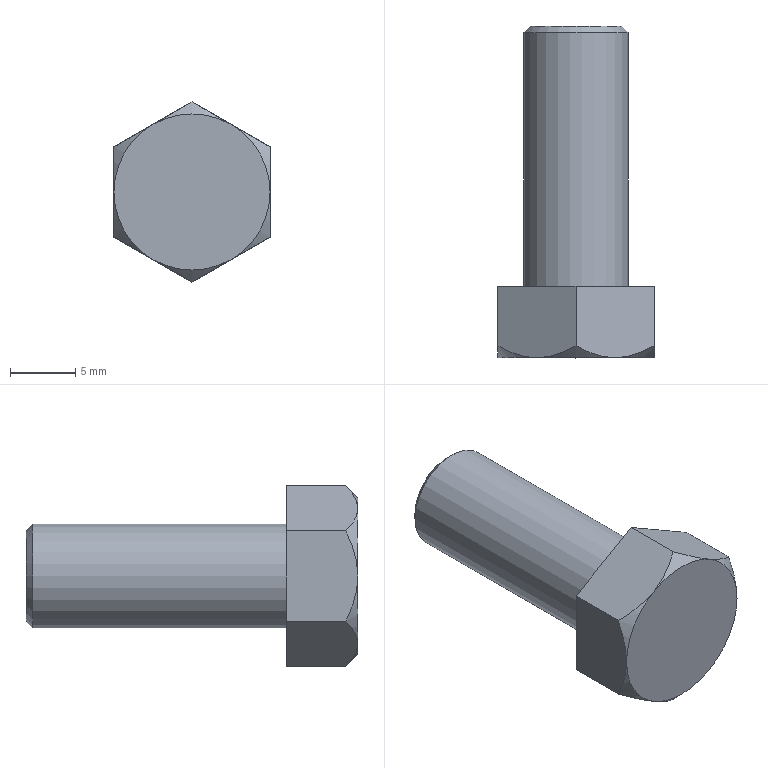Component | NX | BOLT_M8X20_3 | 1 solid | 17 faces | volume 1685 mm3 | plane 9 | cone 7 | cylinder 1 | commonest cylinder face diameters 8 x1